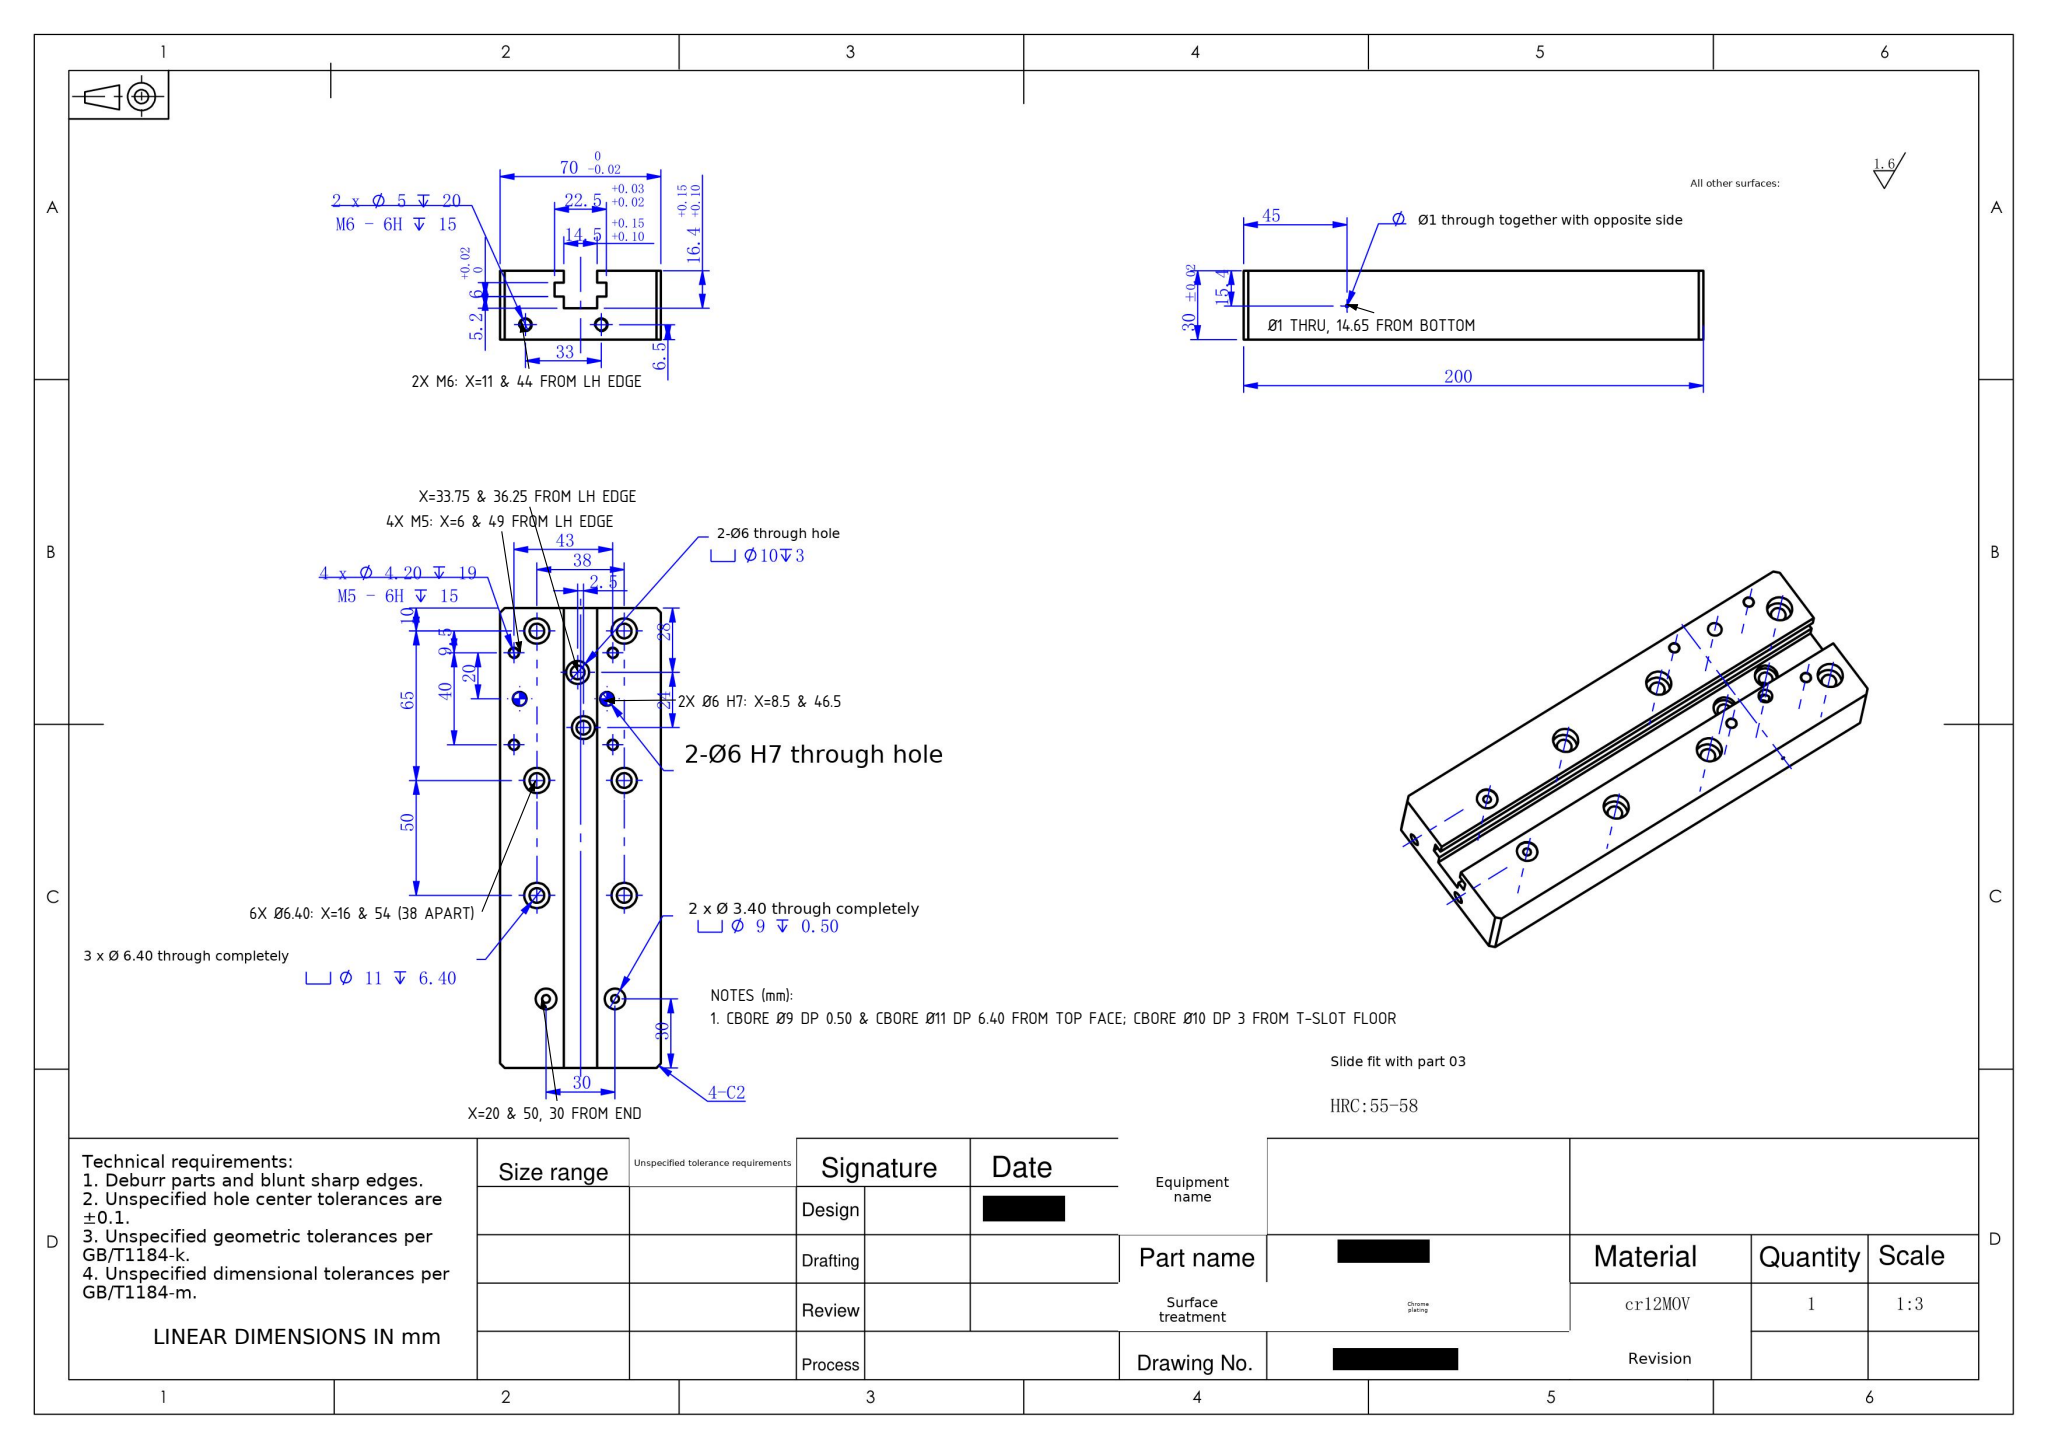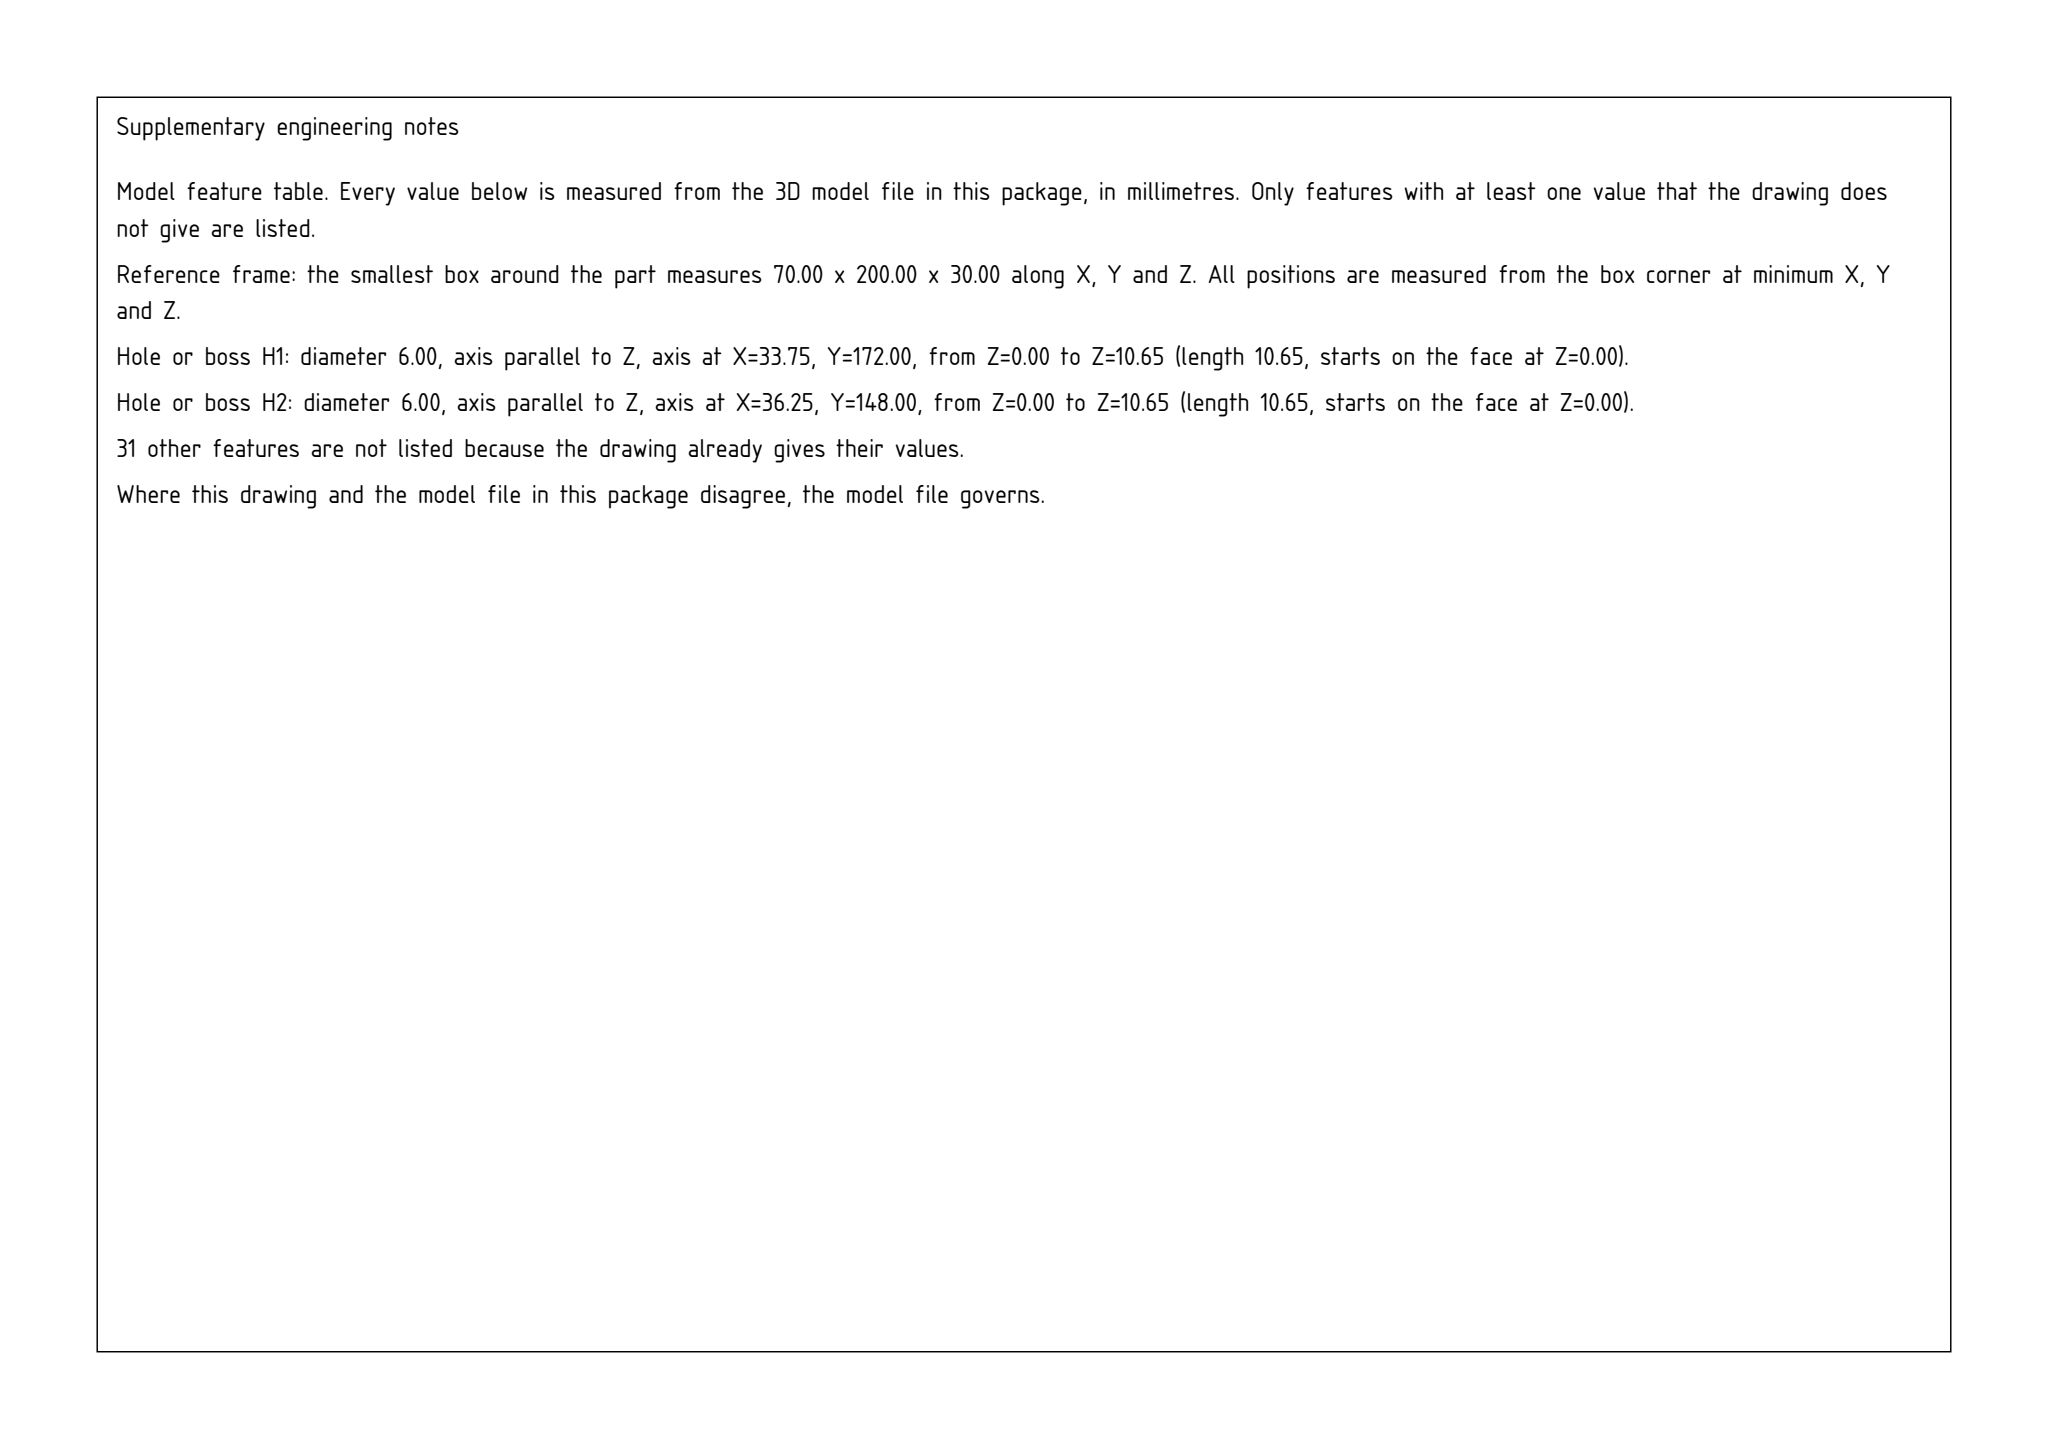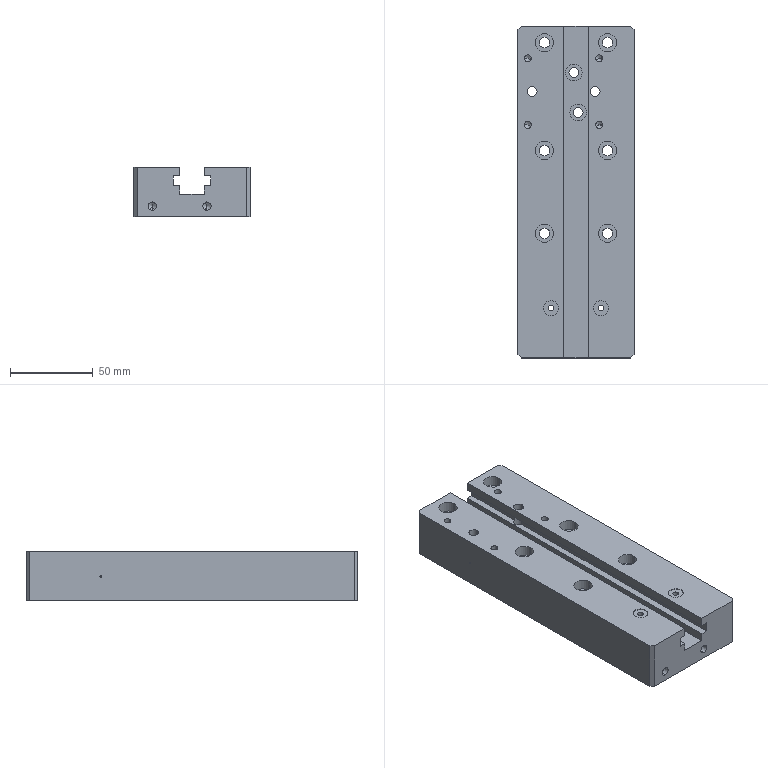Part | SolidWorks | mm | material cr12MOV | 1 solid | 105 faces | box 70 x 200 x 30 mm | volume 349322 mm3 | cylinder 60 | plane 33 | cone 12 | commonest cylinder face diameters 11 x12 6.4 x12 6 x8 4.2 x8 9 x4 3.4 x4 1 x4 10 x4
Drawing notes:
4x M5-6H HOLES AT 6 & 49 FROM LEFT EDGE OF 70 WIDTH | from the solid: Ø4.2 z-holes at x=6.0 and x=49.0 (bbox width 70); y=140.5/180.5
2x Ø6 H7 THRU AT 8.5 & 46.5 FROM LEFT EDGE OF 70 WIDTH | from the solid: Ø6 z-cyls len 30 at x=8.5 and x=46.5, y=160.5
6x Ø6.40 W/ CBORE Ø11 DP 6.40 AT 16 & 54 FROM LEFT EDGE (38 APART) | from the solid: Ø6.4/Ø11 z-holes at x=16.0 and x=54.0; y=75,125,190
2x Ø5 DP 20 / M6-6H DP 15 AT 11 & 44 FROM LEFT EDGE, END FACE | from the solid: Ø5 y-axis holes at x=11.0 and x=44.0, z=6.5, len 20
2x Ø3.40 W/ CBORE Ø9 DP 0.50 AT 20 & 50 FROM LEFT EDGE, 30 FROM END | from the solid: Ø3.4/Ø9 z-holes at x=20.0 & 50.0, y=30.0
CBORE Ø9 DP 0.50 & CBORE Ø11 DP 6.40 FROM TOP FACE; CBORE Ø10 DP 3 FROM T-SLOT FLOOR | from the solid: Ø9 c'bore plane z=29.5 & Ø11 plane z=23.6 (top z=30); Ø10↧3 from slot floor z=13.65 down to 10.65
2-Ø6 DP Ø10 DP 3: X=33.75 (28 END) & 36.25 FROM LH 70 EDGE | from the solid: Ø6/Ø10 CB cyls at [33.75,172] and [36.25,148]; bbox X=70, Y=200 (28 from Y=200 end, 24 apart)
Ø1 CROSS HOLE C/L 14.65 FROM BOTTOM FACE (NOT 15) | from the solid: Ø1 x-axis cyl at z=14.65, y=155; bbox Z=30
build123d program:
from build123d import *

# Parameters (mm, degrees)
SKETCH1_W                                           = 70
SKETCH1_H                                           = 200
BOSS_EXTRUDE1_DEPTH                                 = 30
SKETCH2_W                                           = 14.5
SKETCH2_H                                           = 16.35
CUT_EXTRUDE1_DEPTH                                  = 224.186
SKETCH4_W                                           = 22.5
SKETCH4_H                                           = 6
CUT_EXTRUDE2_DEPTH                                  = 224.186
M6_TAPPED_HOLE1_D                                   = 5
M6_TAPPED_HOLE1_DEPTH                               = 20
M6_TAPPED_HOLE1_TIP                                 = 1.502
M5_TAPPED_HOLE1_D                                   = 4.2
M5_TAPPED_HOLE1_DEPTH                               = 19
M5_TAPPED_HOLE1_TIP                                 = 1.262
SKETCH10_R                                          = 5
CUT_EXTRUDE4_DEPTH                                  = 3
SKETCH11_R                                          = 3
CUT_EXTRUDE5_DEPTH                                  = 169.593
SKETCH12_R                                          = 3
CUT_EXTRUDE6_DEPTH                                  = 171.145
M6_HEX_SOCKET_HEAD_CAP_SCREW_CBORE1_D               = 6.4
M6_HEX_SOCKET_HEAD_CAP_SCREW_CBORE1_CBORE_D         = 11
M6_HEX_SOCKET_HEAD_CAP_SCREW_CBORE1_CBORE_DEPTH     = 6.4
SKETCH15_R                                          = 0.5
CUT_EXTRUDE7_DEPTH                                  = 158.916
CHAMFER1_SIZE                                       = 2
CYLINDRICAL_COUNTERSUNK_HOLE_FOR_M3_HEX_D           = 3.4
CYLINDRICAL_COUNTERSUNK_HOLE_FOR_M3_HEX_CBORE_D     = 9
CYLINDRICAL_COUNTERSUNK_HOLE_FOR_M3_HEX_CBORE_DEPTH = 0.5


with BuildPart() as part:
    # Sketch1 → Boss-Extrude1 (new body)
    with BuildSketch(Plane.XY):
        with Locations((-59.402, -38.338)):
            Rectangle(SKETCH1_W, SKETCH1_H)
    extrude(amount=BOSS_EXTRUDE1_DEPTH)

    # Sketch2 → Cut-Extrude1 (cut, through all)
    with BuildSketch(Plane(origin=(0, -138.338, 0), x_dir=(-1, 0, 0), z_dir=(0, -1, 0))):
        with Locations((59.402, -21.825)):
            Rectangle(SKETCH2_W, SKETCH2_H)
    extrude(amount=-CUT_EXTRUDE1_DEPTH, mode=Mode.SUBTRACT)

    # Sketch4 → Cut-Extrude2 (cut, through all)
    with BuildSketch(Plane(origin=(0, 61.662, 0), x_dir=(1, 0, 0), z_dir=(0, 1, 0))):
        with Locations((-59.402, -21.8)):
            Rectangle(SKETCH4_W, SKETCH4_H)
    extrude(amount=-CUT_EXTRUDE2_DEPTH, mode=Mode.SUBTRACT)

    # M6 Tapped Hole1
    with Locations(Plane(origin=(0, -138.338, 0), x_dir=(-1, 0, 0), z_dir=(0, -1, 0))):
        with Locations((83.402, -6.5), (50.402, -6.5)):
            Hole(M6_TAPPED_HOLE1_D / 2, depth=M6_TAPPED_HOLE1_DEPTH)
            with Locations((0, 0, -(M6_TAPPED_HOLE1_DEPTH + M6_TAPPED_HOLE1_TIP / 2))):  # 118° drill point
                Cone(0, M6_TAPPED_HOLE1_D / 2, M6_TAPPED_HOLE1_TIP, mode=Mode.SUBTRACT)

    # M5 Tapped Hole1
    with Locations(Plane.XY.offset(30)):
        with Locations((-88.402, 2.162), (-88.402, 42.162), (-45.402, 42.162), (-45.402, 2.162)):
            Hole(M5_TAPPED_HOLE1_D / 2, depth=M5_TAPPED_HOLE1_DEPTH)
            with Locations((0, 0, -(M5_TAPPED_HOLE1_DEPTH + M5_TAPPED_HOLE1_TIP / 2))):  # 118° drill point
                Cone(0, M5_TAPPED_HOLE1_D / 2, M5_TAPPED_HOLE1_TIP, mode=Mode.SUBTRACT)

    # Sketch10 → Cut-Extrude4 (cut)
    with BuildSketch(Plane.XY.offset(13.65)):
        with Locations((-58.152, 9.662)):
            Circle(SKETCH10_R)
        with Locations((-60.652, 33.662)):
            Circle(SKETCH10_R)
    extrude(amount=-CUT_EXTRUDE4_DEPTH, mode=Mode.SUBTRACT)

    # Sketch11 → Cut-Extrude5 (cut, through all)
    with BuildSketch(Plane.XY.offset(10.65)):
        with Locations((-58.152, 9.662)):
            Circle(SKETCH11_R)
        with Locations((-60.652, 33.662)):
            Circle(SKETCH11_R)
    extrude(amount=-CUT_EXTRUDE5_DEPTH, mode=Mode.SUBTRACT)

    # Sketch12 → Cut-Extrude6 (cut, through all)
    with BuildSketch(Plane.XY.offset(30)):
        with Locations((-47.902, 22.162)):
            Circle(SKETCH12_R)
        with Locations((-85.902, 22.162)):
            Circle(SKETCH12_R)
    extrude(amount=-CUT_EXTRUDE6_DEPTH, mode=Mode.SUBTRACT)

    # M6 Hex Socket Head Cap Screw CBORE1 (through all)
    with Locations(Plane.XY.offset(30)):
        with Locations((-40.402, 51.662), (-40.402, -13.338), (-40.402, -63.338)):
            m6_hex_socket_head_cap_screw_cbore1 = CounterBoreHole(M6_HEX_SOCKET_HEAD_CAP_SCREW_CBORE1_D / 2, M6_HEX_SOCKET_HEAD_CAP_SCREW_CBORE1_CBORE_D / 2, M6_HEX_SOCKET_HEAD_CAP_SCREW_CBORE1_CBORE_DEPTH)

    # Mirror1: M6 Hex Socket Head Cap Screw CBORE1 across plane
    add(m6_hex_socket_head_cap_screw_cbore1.mirror(Plane(origin=(-59.402, 0, 0), x_dir=(0, 0, 1), z_dir=(1, 0, 0))), mode=Mode.SUBTRACT)

    # Sketch15 → Cut-Extrude7 (cut, through all)
    with BuildSketch(Plane(origin=(-24.402, 0, 0), x_dir=(0, 0, -1), z_dir=(1, 0, 0))):
        with Locations(Location((-14.65, 16.662, 0), (0, 0, 90))):
            Circle(SKETCH15_R)
    extrude(amount=-CUT_EXTRUDE7_DEPTH, mode=Mode.SUBTRACT)

    # Chamfer1
    chamfer1_edges = [part.edges().sort_by_distance(p)[0] for p in [
        (-94.402, 61.662, 15),
        (-24.402, 61.662, 15),
        (-24.402, -138.338, 15),
        (-94.402, -138.338, 15),
    ]]
    chamfer(chamfer1_edges, length=CHAMFER1_SIZE)

    # Cylindrical Countersunk Hole for M3 Hex (through all)
    with Locations(Plane.XY.offset(30)):
        with Locations((-74.402, -108.338), (-44.402, -108.338)):
            CounterBoreHole(CYLINDRICAL_COUNTERSUNK_HOLE_FOR_M3_HEX_D / 2, CYLINDRICAL_COUNTERSUNK_HOLE_FOR_M3_HEX_CBORE_D / 2, CYLINDRICAL_COUNTERSUNK_HOLE_FOR_M3_HEX_CBORE_DEPTH)


solid = part.part